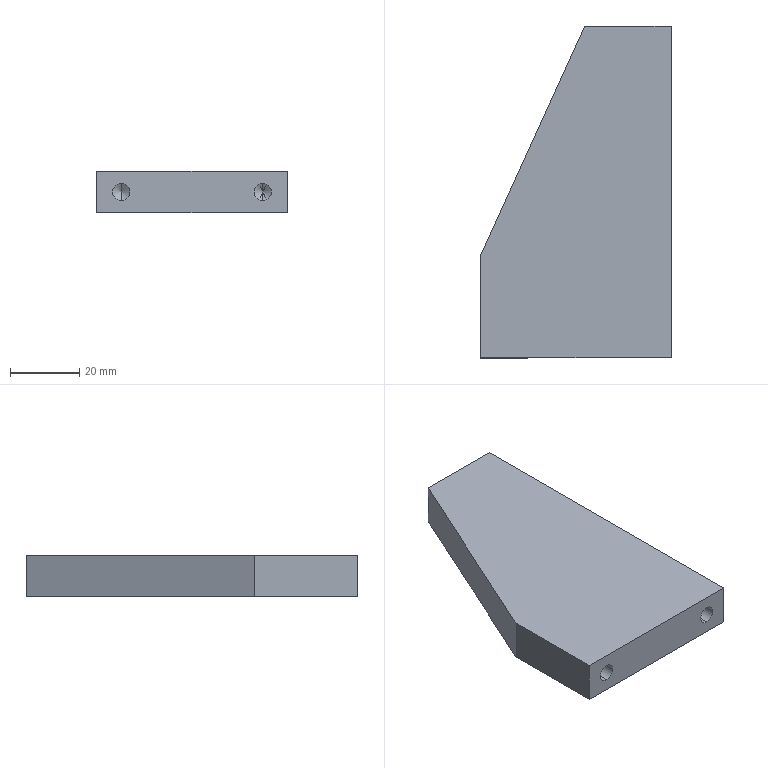Component | SolidWorks | ClampingAssembly-1_A83-1 | 1 solid | 23 faces | box 55 x 96 x 12 mm | volume 50263 mm3 | cylinder 8 | cone 8 | plane 7 | commonest cylinder face diameters 5 x8 | material A6061
build123d program:
from build123d import *

# Parameters (mm, degrees)
SKETCH1_W             = 96
SKETCH1_H             = 55
BOSS_EXTRUDE1_DEPTH   = 6
CUT_EXTRUDE1_DEPTH    = 57.606
M6_TAPPED_HOLE1_D     = 5
M6_TAPPED_HOLE1_DEPTH = 15
M6_TAPPED_HOLE1_TIP   = 1.502
M6_TAPPED_HOLE2_D     = 5
M6_TAPPED_HOLE2_DEPTH = 15
M6_TAPPED_HOLE2_TIP   = 1.502


with BuildPart() as part:
    # Sketch1 → Boss-Extrude1 (new, symmetric)
    with BuildSketch(Plane(origin=(0, 0, 0), x_dir=(0, 0, -1), z_dir=(1, 0, 0))):
        Rectangle(SKETCH1_W, SKETCH1_H)
    extrude(amount=BOSS_EXTRUDE1_DEPTH, both=True)

    # Sketch2 → Cut-Extrude1 (cut, through all)
    with BuildSketch(Plane(origin=(6, 0, 0), x_dir=(0, 0, -1), z_dir=(1, 0, 0))):
        Polygon((48, 27.5), (-18, 27.5), (48, -2.5), align=None)
    extrude(amount=-CUT_EXTRUDE1_DEPTH, mode=Mode.SUBTRACT)

    # M6 Tapped Hole1
    with Locations(Plane.XY.offset(48)):
        with Locations((0, -20.5), (0, 20.5)):
            Hole(M6_TAPPED_HOLE1_D / 2, depth=M6_TAPPED_HOLE1_DEPTH)
            with Locations((0, 0, -(M6_TAPPED_HOLE1_DEPTH + M6_TAPPED_HOLE1_TIP / 2))):  # 118° drill point
                Cone(0, M6_TAPPED_HOLE1_D / 2, M6_TAPPED_HOLE1_TIP, mode=Mode.SUBTRACT)

    # M6 Tapped Hole2
    with Locations(Plane(origin=(0, -27.5, 0), x_dir=(-1, 0, 0), z_dir=(0, -1, 0))):
        with Locations((0, -22), (0, 38)):
            Hole(M6_TAPPED_HOLE2_D / 2, depth=M6_TAPPED_HOLE2_DEPTH)
            with Locations((0, 0, -(M6_TAPPED_HOLE2_DEPTH + M6_TAPPED_HOLE2_TIP / 2))):  # 118° drill point
                Cone(0, M6_TAPPED_HOLE2_D / 2, M6_TAPPED_HOLE2_TIP, mode=Mode.SUBTRACT)


solid = part.part

# Placed as in the assembly
solid = solid.moved(Location((-57.051, 24.036, -0.5), (90, 0, 90)))
STEP:
#1=COLOUR_RGB('',0.7922,0.8196,0.9333);
#2=FILL_AREA_STYLE_COLOUR('',#1);
#3=FILL_AREA_STYLE('',(#2));
#4=SURFACE_STYLE_FILL_AREA(#3);
#5=SURFACE_SIDE_STYLE('',(#4));
#6=SURFACE_STYLE_USAGE(.BOTH.,#5);
#7=PRESENTATION_STYLE_ASSIGNMENT((#6));
#8=CARTESIAN_POINT('',(-1.754,-0.01828,-0.01969));
#9=VERTEX_POINT('',#8);
#10=CARTESIAN_POINT('',(-1.754,0.1786,-0.01969));
#11=VERTEX_POINT('',#10);
#12=CARTESIAN_POINT('',(-1.754,0.08015,-0.01969));
#13=DIRECTION('',(1.,0.,0.));
#14=DIRECTION('',(0.,1.,0.));
#15=AXIS2_PLACEMENT_3D('',#12,#13,#14);
#16=CIRCLE('',#15,0.09843);
#17=EDGE_CURVE('',#9,#11,#16,.T.);
#18=ORIENTED_EDGE('',*,*,#17,.F.);
#19=CARTESIAN_POINT('',(-1.163,-0.01828,-0.01969));
#20=VERTEX_POINT('',#19);
#21=CARTESIAN_POINT('',(-1.163,-0.01828,-0.01969));
#22=DIRECTION('',(1.,0.,0.));
#23=VECTOR('',#22,39.37);
#24=LINE('',#21,#23);
#25=EDGE_CURVE('',#9,#20,#24,.T.);
#26=ORIENTED_EDGE('',*,*,#25,.T.);
#27=CARTESIAN_POINT('',(-1.163,0.1786,-0.01969));
#28=VERTEX_POINT('',#27);
#29=CARTESIAN_POINT('',(-1.163,0.08015,-0.01969));
#30=DIRECTION('',(1.,0.,0.));
#31=DIRECTION('',(0.,1.,0.));
#32=AXIS2_PLACEMENT_3D('',#29,#30,#31);
#33=CIRCLE('',#32,0.09843);
#34=EDGE_CURVE('',#20,#28,#33,.T.);
#35=ORIENTED_EDGE('',*,*,#34,.T.);
#36=CARTESIAN_POINT('',(-1.163,0.1786,-0.01969));
#37=DIRECTION('',(1.,0.,0.));
#38=VECTOR('',#37,39.37);
#39=LINE('',#36,#38);
#40=EDGE_CURVE('',#11,#28,#39,.T.);
#41=ORIENTED_EDGE('',*,*,#40,.F.);
#42=EDGE_LOOP('',(#18,#26,#35,#41));
#43=FACE_OUTER_BOUND('',#42,.T.);
#44=CARTESIAN_POINT('',(-1.163,0.08015,-0.01969));
#45=DIRECTION('',(1.,0.,0.));
#46=DIRECTION('',(0.,1.,0.));
#47=AXIS2_PLACEMENT_3D('',#44,#45,#46);
#48=CYLINDRICAL_SURFACE('',#47,0.09843);
#49=ADVANCED_FACE('',(#43),#48,.F.);
#50=CARTESIAN_POINT('',(-1.813,0.08015,-0.01969));
#51=VERTEX_POINT('',#50);
#52=CARTESIAN_POINT('',(-1.754,0.1786,-0.01969));
#53=DIRECTION('',(0.515,0.8572,0.));
#54=VECTOR('',#53,39.37);
#55=LINE('',#52,#54);
#56=EDGE_CURVE('',#51,#11,#55,.T.);
#57=ORIENTED_EDGE('',*,*,#56,.F.);
#58=CARTESIAN_POINT('',(-1.754,-0.01828,-0.01969));
#59=DIRECTION('',(0.515,-0.8572,-0.));
#60=VECTOR('',#59,39.37);
#61=LINE('',#58,#60);
#62=EDGE_CURVE('',#51,#9,#61,.T.);
#63=ORIENTED_EDGE('',*,*,#62,.T.);
#64=ORIENTED_EDGE('',*,*,#17,.T.);
#65=EDGE_LOOP('',(#57,#63,#64));
#66=FACE_OUTER_BOUND('',#65,.T.);
#67=CARTESIAN_POINT('',(-1.754,0.08015,-0.01969));
#68=DIRECTION('',(1.,0.,0.));
#69=DIRECTION('',(0.,1.,0.));
#70=AXIS2_PLACEMENT_3D('',#67,#68,#69);
#71=CONICAL_SURFACE('',#70,0.09843,1.03);
#72=ADVANCED_FACE('',(#66),#71,.F.);
#73=CARTESIAN_POINT('',(-1.754,2.344,-0.01969));
#74=VERTEX_POINT('',#73);
#75=CARTESIAN_POINT('',(-1.754,2.541,-0.01969));
#76=VERTEX_POINT('',#75);
#77=CARTESIAN_POINT('',(-1.754,2.442,-0.01969));
#78=DIRECTION('',(1.,0.,0.));
#79=DIRECTION('',(0.,1.,0.));
#80=AXIS2_PLACEMENT_3D('',#77,#78,#79);
#81=CIRCLE('',#80,0.09843);
#82=EDGE_CURVE('',#74,#76,#81,.T.);
#83=ORIENTED_EDGE('',*,*,#82,.F.);
#84=CARTESIAN_POINT('',(-1.163,2.344,-0.01969));
#85=VERTEX_POINT('',#84);
#86=CARTESIAN_POINT('',(-1.163,2.344,-0.01969));
#87=DIRECTION('',(1.,0.,0.));
#88=VECTOR('',#87,39.37);
#89=LINE('',#86,#88);
#90=EDGE_CURVE('',#74,#85,#89,.T.);
#91=ORIENTED_EDGE('',*,*,#90,.T.);
#92=CARTESIAN_POINT('',(-1.163,2.541,-0.01969));
#93=VERTEX_POINT('',#92);
#94=CARTESIAN_POINT('',(-1.163,2.442,-0.01969));
#95=DIRECTION('',(1.,0.,0.));
#96=DIRECTION('',(0.,1.,0.));
#97=AXIS2_PLACEMENT_3D('',#94,#95,#96);
#98=CIRCLE('',#97,0.09843);
#99=EDGE_CURVE('',#85,#93,#98,.T.);
#100=ORIENTED_EDGE('',*,*,#99,.T.);
#101=CARTESIAN_POINT('',(-1.163,2.541,-0.01969));
#102=DIRECTION('',(1.,0.,0.));
#103=VECTOR('',#102,39.37);
#104=LINE('',#101,#103);
#105=EDGE_CURVE('',#76,#93,#104,.T.);
#106=ORIENTED_EDGE('',*,*,#105,.F.);
#107=EDGE_LOOP('',(#83,#91,#100,#106));
#108=FACE_OUTER_BOUND('',#107,.T.);
#109=CARTESIAN_POINT('',(-1.163,2.442,-0.01969));
#110=DIRECTION('',(1.,0.,0.));
#111=DIRECTION('',(0.,1.,0.));
#112=AXIS2_PLACEMENT_3D('',#109,#110,#111);
#113=CYLINDRICAL_SURFACE('',#112,0.09843);
#114=ADVANCED_FACE('',(#108),#113,.F.);
#115=CARTESIAN_POINT('',(-1.813,2.442,-0.01969));
#116=VERTEX_POINT('',#115);
#117=CARTESIAN_POINT('',(-1.754,2.541,-0.01969));
#118=DIRECTION('',(0.515,0.8572,0.));
#119=VECTOR('',#118,39.37);
#120=LINE('',#117,#119);
#121=EDGE_CURVE('',#116,#76,#120,.T.);
#122=ORIENTED_EDGE('',*,*,#121,.F.);
#123=CARTESIAN_POINT('',(-1.754,2.344,-0.01969));
#124=DIRECTION('',(0.515,-0.8572,-0.));
#125=VECTOR('',#124,39.37);
#126=LINE('',#123,#125);
#127=EDGE_CURVE('',#116,#74,#126,.T.);
#128=ORIENTED_EDGE('',*,*,#127,.T.);
#129=ORIENTED_EDGE('',*,*,#82,.T.);
#130=EDGE_LOOP('',(#122,#128,#129));
#131=FACE_OUTER_BOUND('',#130,.T.);
#132=CARTESIAN_POINT('',(-1.754,2.442,-0.01969));
#133=DIRECTION('',(1.,0.,0.));
#134=DIRECTION('',(0.,1.,0.));
#135=AXIS2_PLACEMENT_3D('',#132,#133,#134);
#136=CONICAL_SURFACE('',#135,0.09843,1.03);
#137=ADVANCED_FACE('',(#131),#136,.F.);
#138=CARTESIAN_POINT('',(-1.439,-0.3529,-0.1181));
#139=VERTEX_POINT('',#138);
#140=CARTESIAN_POINT('',(-1.439,-0.3529,0.07874));
#141=VERTEX_POINT('',#140);
#142=CARTESIAN_POINT('',(-1.439,-0.3529,-0.01969));
#143=DIRECTION('',(0.,-1.,-0.));
#144=DIRECTION('',(0.,-0.,1.));
#145=AXIS2_PLACEMENT_3D('',#142,#143,#144);
#146=CIRCLE('',#145,0.09843);
#147=EDGE_CURVE('',#139,#141,#146,.T.);
#148=ORIENTED_EDGE('',*,*,#147,.F.);
#149=CARTESIAN_POINT('',(-1.439,-0.9435,-0.1181));
#150=VERTEX_POINT('',#149);
#151=CARTESIAN_POINT('',(-1.439,-0.9435,-0.1181));
#152=DIRECTION('',(0.,-1.,-0.));
#153=VECTOR('',#152,39.37);
#154=LINE('',#151,#153);
#155=EDGE_CURVE('',#139,#150,#154,.T.);
#156=ORIENTED_EDGE('',*,*,#155,.T.);
#157=CARTESIAN_POINT('',(-1.439,-0.9435,0.07874));
#158=VERTEX_POINT('',#157);
#159=CARTESIAN_POINT('',(-1.439,-0.9435,-0.01969));
#160=DIRECTION('',(0.,-1.,-0.));
#161=DIRECTION('',(0.,-0.,1.));
#162=AXIS2_PLACEMENT_3D('',#159,#160,#161);
#163=CIRCLE('',#162,0.09843);
#164=EDGE_CURVE('',#150,#158,#163,.T.);
#165=ORIENTED_EDGE('',*,*,#164,.T.);
#166=CARTESIAN_POINT('',(-1.439,-0.9435,0.07874));
#167=DIRECTION('',(0.,-1.,-0.));
#168=VECTOR('',#167,39.37);
#169=LINE('',#166,#168);
#170=EDGE_CURVE('',#141,#158,#169,.T.);
#171=ORIENTED_EDGE('',*,*,#170,.F.);
#172=EDGE_LOOP('',(#148,#156,#165,#171));
#173=FACE_OUTER_BOUND('',#172,.T.);
#174=CARTESIAN_POINT('',(-1.439,-0.9435,-0.01969));
#175=DIRECTION('',(0.,-1.,-0.));
#176=DIRECTION('',(0.,-0.,1.));
#177=AXIS2_PLACEMENT_3D('',#174,#175,#176);
#178=CYLINDRICAL_SURFACE('',#177,0.09843);
#179=ADVANCED_FACE('',(#173),#178,.F.);
#180=CARTESIAN_POINT('',(-1.439,-0.2938,-0.01969));
#181=VERTEX_POINT('',#180);
#182=CARTESIAN_POINT('',(-1.439,-0.3529,0.07874));
#183=DIRECTION('',(-0.,-0.515,0.8572));
#184=VECTOR('',#183,39.37);
#185=LINE('',#182,#184);
#186=EDGE_CURVE('',#181,#141,#185,.T.);
#187=ORIENTED_EDGE('',*,*,#186,.F.);
#188=CARTESIAN_POINT('',(-1.439,-0.3529,-0.1181));
#189=DIRECTION('',(0.,-0.515,-0.8572));
#190=VECTOR('',#189,39.37);
#191=LINE('',#188,#190);
#192=EDGE_CURVE('',#181,#139,#191,.T.);
#193=ORIENTED_EDGE('',*,*,#192,.T.);
#194=ORIENTED_EDGE('',*,*,#147,.T.);
#195=EDGE_LOOP('',(#187,#193,#194));
#196=FACE_OUTER_BOUND('',#195,.T.);
#197=CARTESIAN_POINT('',(-1.439,-0.3529,-0.01969));
#198=DIRECTION('',(0.,-1.,-0.));
#199=DIRECTION('',(0.,-0.,1.));
#200=AXIS2_PLACEMENT_3D('',#197,#198,#199);
#201=CONICAL_SURFACE('',#200,0.09843,1.03);
#202=ADVANCED_FACE('',(#196),#201,.F.);
#203=CARTESIAN_POINT('',(-3.053,-0.3529,-0.1181));
#204=VERTEX_POINT('',#203);
#205=CARTESIAN_POINT('',(-3.053,-0.3529,0.07874));
#206=VERTEX_POINT('',#205);
#207=CARTESIAN_POINT('',(-3.053,-0.3529,-0.01969));
#208=DIRECTION('',(0.,-1.,-0.));
#209=DIRECTION('',(0.,-0.,1.));
#210=AXIS2_PLACEMENT_3D('',#207,#208,#209);
#211=CIRCLE('',#210,0.09843);
#212=EDGE_CURVE('',#204,#206,#211,.T.);
#213=ORIENTED_EDGE('',*,*,#212,.F.);
#214=CARTESIAN_POINT('',(-3.053,-0.9435,-0.1181));
#215=VERTEX_POINT('',#214);
#216=CARTESIAN_POINT('',(-3.053,-0.9435,-0.1181));
#217=DIRECTION('',(0.,-1.,-0.));
#218=VECTOR('',#217,39.37);
#219=LINE('',#216,#218);
#220=EDGE_CURVE('',#204,#215,#219,.T.);
#221=ORIENTED_EDGE('',*,*,#220,.T.);
#222=CARTESIAN_POINT('',(-3.053,-0.9435,0.07874));
#223=VERTEX_POINT('',#222);
#224=CARTESIAN_POINT('',(-3.053,-0.9435,-0.01969));
#225=DIRECTION('',(0.,-1.,-0.));
#226=DIRECTION('',(0.,-0.,1.));
#227=AXIS2_PLACEMENT_3D('',#224,#225,#226);
#228=CIRCLE('',#227,0.09843);
#229=EDGE_CURVE('',#215,#223,#228,.T.);
#230=ORIENTED_EDGE('',*,*,#229,.T.);
#231=CARTESIAN_POINT('',(-3.053,-0.9435,0.07874));
#232=DIRECTION('',(0.,-1.,-0.));
#233=VECTOR('',#232,39.37);
#234=LINE('',#231,#233);
#235=EDGE_CURVE('',#206,#223,#234,.T.);
#236=ORIENTED_EDGE('',*,*,#235,.F.);
#237=EDGE_LOOP('',(#213,#221,#230,#236));
#238=FACE_OUTER_BOUND('',#237,.T.);
#239=CARTESIAN_POINT('',(-3.053,-0.9435,-0.01969));
#240=DIRECTION('',(0.,-1.,-0.));
#241=DIRECTION('',(0.,-0.,1.));
#242=AXIS2_PLACEMENT_3D('',#239,#240,#241);
#243=CYLINDRICAL_SURFACE('',#242,0.09843);
#244=ADVANCED_FACE('',(#238),#243,.F.);
#245=CARTESIAN_POINT('',(-3.053,-0.2938,-0.01969));
#246=VERTEX_POINT('',#245);
#247=CARTESIAN_POINT('',(-3.053,-0.3529,0.07874));
#248=DIRECTION('',(-0.,-0.515,0.8572));
#249=VECTOR('',#248,39.37);
#250=LINE('',#247,#249);
#251=EDGE_CURVE('',#246,#206,#250,.T.);
#252=ORIENTED_EDGE('',*,*,#251,.F.);
#253=CARTESIAN_POINT('',(-3.053,-0.3529,-0.1181));
#254=DIRECTION('',(0.,-0.515,-0.8572));
#255=VECTOR('',#254,39.37);
#256=LINE('',#253,#255);
#257=EDGE_CURVE('',#246,#204,#256,.T.);
#258=ORIENTED_EDGE('',*,*,#257,.T.);
#259=ORIENTED_EDGE('',*,*,#212,.T.);
#260=EDGE_LOOP('',(#252,#258,#259));
#261=FACE_OUTER_BOUND('',#260,.T.);
#262=CARTESIAN_POINT('',(-3.053,-0.3529,-0.01969));
#263=DIRECTION('',(0.,-1.,-0.));
#264=DIRECTION('',(0.,-0.,1.));
#265=AXIS2_PLACEMENT_3D('',#262,#263,#264);
#266=CONICAL_SURFACE('',#265,0.09843,1.03);
#267=ADVANCED_FACE('',(#261),#266,.F.);
#268=CARTESIAN_POINT('',(-1.163,2.836,-0.2559));
#269=VERTEX_POINT('',#268);
#270=CARTESIAN_POINT('',(-2.148,2.836,-0.2559));
#271=VERTEX_POINT('',#270);
#272=CARTESIAN_POINT('',(-3.329,2.836,-0.2559));
#273=DIRECTION('',(-1.,-0.,-0.));
#274=VECTOR('',#273,39.37);
#275=LINE('',#272,#274);
#276=EDGE_CURVE('',#269,#271,#275,.T.);
#277=ORIENTED_EDGE('',*,*,#276,.T.);
#278=CARTESIAN_POINT('',(-2.148,2.836,0.2165));
#279=VERTEX_POINT('',#278);
#280=CARTESIAN_POINT('',(-2.148,2.836,-0.2559));
#281=DIRECTION('',(-0.,-0.,1.));
#282=VECTOR('',#281,39.37);
#283=LINE('',#280,#282);
#284=EDGE_CURVE('',#271,#279,#283,.T.);
#285=ORIENTED_EDGE('',*,*,#284,.T.);
#286=CARTESIAN_POINT('',(-1.163,2.836,0.2165));
#287=VERTEX_POINT('',#286);
#288=CARTESIAN_POINT('',(-3.329,2.836,0.2165));
#289=DIRECTION('',(-1.,-0.,-0.));
#290=VECTOR('',#289,39.37);
#291=LINE('',#288,#290);
#292=EDGE_CURVE('',#287,#279,#291,.T.);
#293=ORIENTED_EDGE('',*,*,#292,.F.);
#294=CARTESIAN_POINT('',(-1.163,2.836,0.2165));
#295=DIRECTION('',(0.,0.,-1.));
#296=VECTOR('',#295,39.37);
#297=LINE('',#294,#296);
#298=EDGE_CURVE('',#287,#269,#297,.T.);
#299=ORIENTED_EDGE('',*,*,#298,.T.);
#300=EDGE_LOOP('',(#277,#285,#293,#299));
#301=FACE_OUTER_BOUND('',#300,.T.);
#302=CARTESIAN_POINT('',(-3.329,2.836,0.2165));
#303=DIRECTION('',(0.,-1.,-0.));
#304=DIRECTION('',(-0.,-0.,1.));
#305=AXIS2_PLACEMENT_3D('',#302,#303,#304);
#306=PLANE('',#305);
#307=ADVANCED_FACE('',(#301),#306,.F.);
#308=CARTESIAN_POINT('',(-3.329,0.2376,0.2165));
#309=VERTEX_POINT('',#308);
#310=CARTESIAN_POINT('',(-3.329,-0.9435,0.2165));
#311=VERTEX_POINT('',#310);
#312=CARTESIAN_POINT('',(-3.329,-0.9435,0.2165));
#313=DIRECTION('',(0.,-1.,-0.));
#314=VECTOR('',#313,39.37);
#315=LINE('',#312,#314);
#316=EDGE_CURVE('',#309,#311,#315,.T.);
#317=ORIENTED_EDGE('',*,*,#316,.F.);
#318=CARTESIAN_POINT('',(-3.329,0.2376,-0.2559));
#319=VERTEX_POINT('',#318);
#320=CARTESIAN_POINT('',(-3.329,0.2376,-0.2559));
#321=DIRECTION('',(-0.,-0.,1.));
#322=VECTOR('',#321,39.37);
#323=LINE('',#320,#322);
#324=EDGE_CURVE('',#319,#309,#323,.T.);
#325=ORIENTED_EDGE('',*,*,#324,.F.);
#326=CARTESIAN_POINT('',(-3.329,-0.9435,-0.2559));
#327=VERTEX_POINT('',#326);
#328=CARTESIAN_POINT('',(-3.329,-0.9435,-0.2559));
#329=DIRECTION('',(0.,-1.,-0.));
#330=VECTOR('',#329,39.37);
#331=LINE('',#328,#330);
#332=EDGE_CURVE('',#319,#327,#331,.T.);
#333=ORIENTED_EDGE('',*,*,#332,.T.);
#334=CARTESIAN_POINT('',(-3.329,-0.9435,0.2165));
#335=DIRECTION('',(0.,0.,-1.));
#336=VECTOR('',#335,39.37);
#337=LINE('',#334,#336);
#338=EDGE_CURVE('',#311,#327,#337,.T.);
#339=ORIENTED_EDGE('',*,*,#338,.F.);
#340=EDGE_LOOP('',(#317,#325,#333,#339));
#341=FACE_OUTER_BOUND('',#340,.T.);
#342=CARTESIAN_POINT('',(-3.329,-0.9435,0.2165));
#343=DIRECTION('',(1.,0.,0.));
#344=DIRECTION('',(-0.,1.,0.));
#345=AXIS2_PLACEMENT_3D('',#342,#343,#344);
#346=PLANE('',#345);
#347=ADVANCED_FACE('',(#341),#346,.F.);
#348=CARTESIAN_POINT('',(-1.439,-0.9435,-0.01969));
#349=DIRECTION('',(0.,-1.,-0.));
#350=DIRECTION('',(0.,-0.,1.));
#351=AXIS2_PLACEMENT_3D('',#348,#349,#350);
#352=CIRCLE('',#351,0.09843);
#353=EDGE_CURVE('',#158,#150,#352,.T.);
#354=ORIENTED_EDGE('',*,*,#353,.F.);
#355=ORIENTED_EDGE('',*,*,#164,.F.);
#356=EDGE_LOOP('',(#354,#355));
#357=FACE_BOUND('',#356,.T.);
#358=CARTESIAN_POINT('',(-3.053,-0.9435,-0.01969));
#359=DIRECTION('',(0.,-1.,-0.));
#360=DIRECTION('',(0.,-0.,1.));
#361=AXIS2_PLACEMENT_3D('',#358,#359,#360);
#362=CIRCLE('',#361,0.09843);
#363=EDGE_CURVE('',#223,#215,#362,.T.);
#364=ORIENTED_EDGE('',*,*,#363,.F.);
#365=ORIENTED_EDGE('',*,*,#229,.F.);
#366=EDGE_LOOP('',(#364,#365));
#367=FACE_BOUND('',#366,.T.);
#368=CARTESIAN_POINT('',(-1.163,-0.9435,-0.2559));
#369=VERTEX_POINT('',#368);
#370=CARTESIAN_POINT('',(-3.329,-0.9435,-0.2559));
#371=DIRECTION('',(1.,0.,0.));
#372=VECTOR('',#371,39.37);
#373=LINE('',#370,#372);
#374=EDGE_CURVE('',#327,#369,#373,.T.);
#375=ORIENTED_EDGE('',*,*,#374,.T.);
#376=CARTESIAN_POINT('',(-1.163,-0.9435,0.2165));
#377=VERTEX_POINT('',#376);
#378=CARTESIAN_POINT('',(-1.163,-0.9435,0.2165));
#379=DIRECTION('',(0.,0.,-1.));
#380=VECTOR('',#379,39.37);
#381=LINE('',#378,#380);
#382=EDGE_CURVE('',#377,#369,#381,.T.);
#383=ORIENTED_EDGE('',*,*,#382,.F.);
#384=CARTESIAN_POINT('',(-3.329,-0.9435,0.2165));
#385=DIRECTION('',(1.,0.,0.));
#386=VECTOR('',#385,39.37);
#387=LINE('',#384,#386);
#388=EDGE_CURVE('',#311,#377,#387,.T.);
#389=ORIENTED_EDGE('',*,*,#388,.F.);
#390=ORIENTED_EDGE('',*,*,#338,.T.);
#391=EDGE_LOOP('',(#375,#383,#389,#390));
#392=FACE_OUTER_BOUND('',#391,.T.);
#393=CARTESIAN_POINT('',(-3.329,-0.9435,0.2165));
#394=DIRECTION('',(-0.,1.,0.));
#395=DIRECTION('',(-1.,-0.,-0.));
#396=AXIS2_PLACEMENT_3D('',#393,#394,#395);
#397=PLANE('',#396);
#398=ADVANCED_FACE('',(#357,#367,#392),#397,.F.);
#399=CARTESIAN_POINT('',(-1.163,0.08015,-0.01969));
#400=DIRECTION('',(1.,0.,0.));
#401=DIRECTION('',(0.,1.,0.));
#402=AXIS2_PLACEMENT_3D('',#399,#400,#401);
#403=CIRCLE('',#402,0.09843);
#404=EDGE_CURVE('',#28,#20,#403,.T.);
#405=ORIENTED_EDGE('',*,*,#404,.F.);
#406=ORIENTED_EDGE('',*,*,#34,.F.);
#407=EDGE_LOOP('',(#405,#406));
#408=FACE_BOUND('',#407,.T.);
#409=CARTESIAN_POINT('',(-1.163,2.442,-0.01969));
#410=DIRECTION('',(1.,0.,0.));
#411=DIRECTION('',(0.,1.,0.));
#412=AXIS2_PLACEMENT_3D('',#409,#410,#411);
#413=CIRCLE('',#412,0.09843);
#414=EDGE_CURVE('',#93,#85,#413,.T.);
#415=ORIENTED_EDGE('',*,*,#414,.F.);
#416=ORIENTED_EDGE('',*,*,#99,.F.);
#417=EDGE_LOOP('',(#415,#416));
#418=FACE_BOUND('',#417,.T.);
#419=CARTESIAN_POINT('',(-1.163,-0.9435,-0.2559));
#420=DIRECTION('',(-0.,1.,0.));
#421=VECTOR('',#420,39.37);
#422=LINE('',#419,#421);
#423=EDGE_CURVE('',#369,#269,#422,.T.);
#424=ORIENTED_EDGE('',*,*,#423,.T.);
#425=ORIENTED_EDGE('',*,*,#298,.F.);
#426=CARTESIAN_POINT('',(-1.163,-0.9435,0.2165));
#427=DIRECTION('',(-0.,1.,0.));
#428=VECTOR('',#427,39.37);
#429=LINE('',#426,#428);
#430=EDGE_CURVE('',#377,#287,#429,.T.);
#431=ORIENTED_EDGE('',*,*,#430,.F.);
#432=ORIENTED_EDGE('',*,*,#382,.T.);
#433=EDGE_LOOP('',(#424,#425,#431,#432));
#434=FACE_OUTER_BOUND('',#433,.T.);
#435=CARTESIAN_POINT('',(-1.163,-0.9435,0.2165));
#436=DIRECTION('',(-1.,-0.,-0.));
#437=DIRECTION('',(0.,-1.,-0.));
#438=AXIS2_PLACEMENT_3D('',#435,#436,#437);
#439=PLANE('',#438);
#440=ADVANCED_FACE('',(#408,#418,#434),#439,.F.);
#441=CARTESIAN_POINT('',(-3.329,0.2376,0.2165));
#442=DIRECTION('',(0.4138,0.9104,0.));
#443=VECTOR('',#442,39.37);
#444=LINE('',#441,#443);
#445=EDGE_CURVE('',#309,#279,#444,.T.);
#446=ORIENTED_EDGE('',*,*,#445,.F.);
#447=ORIENTED_EDGE('',*,*,#316,.T.);
#448=ORIENTED_EDGE('',*,*,#388,.T.);
#449=ORIENTED_EDGE('',*,*,#430,.T.);
#450=ORIENTED_EDGE('',*,*,#292,.T.);
#451=EDGE_LOOP('',(#446,#447,#448,#449,#450));
#452=FACE_OUTER_BOUND('',#451,.T.);
#453=CARTESIAN_POINT('',(-2.246,0.9463,0.2165));
#454=DIRECTION('',(-0.,-0.,1.));
#455=DIRECTION('',(-0.,1.,0.));
#456=AXIS2_PLACEMENT_3D('',#453,#454,#455);
#457=PLANE('',#456);
#458=ADVANCED_FACE('',(#452),#457,.T.);
#459=ORIENTED_EDGE('',*,*,#332,.F.);
#460=CARTESIAN_POINT('',(-3.329,0.2376,-0.2559));
#461=DIRECTION('',(0.4138,0.9104,0.));
#462=VECTOR('',#461,39.37);
#463=LINE('',#460,#462);
#464=EDGE_CURVE('',#319,#271,#463,.T.);
#465=ORIENTED_EDGE('',*,*,#464,.T.);
#466=ORIENTED_EDGE('',*,*,#276,.F.);
#467=ORIENTED_EDGE('',*,*,#423,.F.);
#468=ORIENTED_EDGE('',*,*,#374,.F.);
#469=EDGE_LOOP('',(#459,#465,#466,#467,#468));
#470=FACE_OUTER_BOUND('',#469,.T.);
#471=CARTESIAN_POINT('',(-2.246,0.9463,-0.2559));
#472=DIRECTION('',(-0.,-0.,1.));
#473=DIRECTION('',(-0.,1.,0.));
#474=AXIS2_PLACEMENT_3D('',#471,#472,#473);
#475=PLANE('',#474);
#476=ADVANCED_FACE('',(#470),#475,.F.);
#477=ORIENTED_EDGE('',*,*,#445,.T.);
#478=ORIENTED_EDGE('',*,*,#284,.F.);
#479=ORIENTED_EDGE('',*,*,#464,.F.);
#480=ORIENTED_EDGE('',*,*,#324,.T.);
#481=EDGE_LOOP('',(#477,#478,#479,#480));
#482=FACE_OUTER_BOUND('',#481,.T.);
#483=CARTESIAN_POINT('',(-3.329,0.2376,-0.2559));
#484=DIRECTION('',(0.9104,-0.4138,-0.));
#485=DIRECTION('',(0.4138,0.9104,0.));
#486=AXIS2_PLACEMENT_3D('',#483,#484,#485);
#487=PLANE('',#486);
#488=ADVANCED_FACE('',(#482),#487,.F.);
#489=ORIENTED_EDGE('',*,*,#257,.F.);
#490=ORIENTED_EDGE('',*,*,#251,.T.);
#491=CARTESIAN_POINT('',(-3.053,-0.3529,-0.01969));
#492=DIRECTION('',(0.,-1.,-0.));
#493=DIRECTION('',(0.,-0.,1.));
#494=AXIS2_PLACEMENT_3D('',#491,#492,#493);
#495=CIRCLE('',#494,0.09843);
#496=EDGE_CURVE('',#206,#204,#495,.T.);
#497=ORIENTED_EDGE('',*,*,#496,.T.);
#498=EDGE_LOOP('',(#489,#490,#497));
#499=FACE_OUTER_BOUND('',#498,.T.);
#500=CARTESIAN_POINT('',(-3.053,-0.3529,-0.01969));
#501=DIRECTION('',(0.,-1.,-0.));
#502=DIRECTION('',(0.,-0.,1.));
#503=AXIS2_PLACEMENT_3D('',#500,#501,#502);
#504=CONICAL_SURFACE('',#503,0.09843,1.03);
#505=ADVANCED_FACE('',(#499),#504,.F.);
#506=ORIENTED_EDGE('',*,*,#220,.F.);
#507=ORIENTED_EDGE('',*,*,#496,.F.);
#508=ORIENTED_EDGE('',*,*,#235,.T.);
#509=ORIENTED_EDGE('',*,*,#363,.T.);
#510=EDGE_LOOP('',(#506,#507,#508,#509));
#511=FACE_OUTER_BOUND('',#510,.T.);
#512=CARTESIAN_POINT('',(-3.053,-0.9435,-0.01969));
#513=DIRECTION('',(0.,-1.,-0.));
#514=DIRECTION('',(0.,-0.,1.));
#515=AXIS2_PLACEMENT_3D('',#512,#513,#514);
#516=CYLINDRICAL_SURFACE('',#515,0.09843);
#517=ADVANCED_FACE('',(#511),#516,.F.);
#518=ORIENTED_EDGE('',*,*,#192,.F.);
#519=ORIENTED_EDGE('',*,*,#186,.T.);
#520=CARTESIAN_POINT('',(-1.439,-0.3529,-0.01969));
#521=DIRECTION('',(0.,-1.,-0.));
#522=DIRECTION('',(0.,-0.,1.));
#523=AXIS2_PLACEMENT_3D('',#520,#521,#522);
#524=CIRCLE('',#523,0.09843);
#525=EDGE_CURVE('',#141,#139,#524,.T.);
#526=ORIENTED_EDGE('',*,*,#525,.T.);
#527=EDGE_LOOP('',(#518,#519,#526));
#528=FACE_OUTER_BOUND('',#527,.T.);
#529=CARTESIAN_POINT('',(-1.439,-0.3529,-0.01969));
#530=DIRECTION('',(0.,-1.,-0.));
#531=DIRECTION('',(0.,-0.,1.));
#532=AXIS2_PLACEMENT_3D('',#529,#530,#531);
#533=CONICAL_SURFACE('',#532,0.09843,1.03);
#534=ADVANCED_FACE('',(#528),#533,.F.);
#535=ORIENTED_EDGE('',*,*,#155,.F.);
#536=ORIENTED_EDGE('',*,*,#525,.F.);
#537=ORIENTED_EDGE('',*,*,#170,.T.);
#538=ORIENTED_EDGE('',*,*,#353,.T.);
#539=EDGE_LOOP('',(#535,#536,#537,#538));
#540=FACE_OUTER_BOUND('',#539,.T.);
#541=CARTESIAN_POINT('',(-1.439,-0.9435,-0.01969));
#542=DIRECTION('',(0.,-1.,-0.));
#543=DIRECTION('',(0.,-0.,1.));
#544=AXIS2_PLACEMENT_3D('',#541,#542,#543);
#545=CYLINDRICAL_SURFACE('',#544,0.09843);
#546=ADVANCED_FACE('',(#540),#545,.F.);
#547=ORIENTED_EDGE('',*,*,#127,.F.);
#548=ORIENTED_EDGE('',*,*,#121,.T.);
#549=CARTESIAN_POINT('',(-1.754,2.442,-0.01969));
#550=DIRECTION('',(1.,0.,0.));
#551=DIRECTION('',(0.,1.,0.));
#552=AXIS2_PLACEMENT_3D('',#549,#550,#551);
#553=CIRCLE('',#552,0.09843);
#554=EDGE_CURVE('',#76,#74,#553,.T.);
#555=ORIENTED_EDGE('',*,*,#554,.T.);
#556=EDGE_LOOP('',(#547,#548,#555));
#557=FACE_OUTER_BOUND('',#556,.T.);
#558=CARTESIAN_POINT('',(-1.754,2.442,-0.01969));
#559=DIRECTION('',(1.,0.,0.));
#560=DIRECTION('',(0.,1.,0.));
#561=AXIS2_PLACEMENT_3D('',#558,#559,#560);
#562=CONICAL_SURFACE('',#561,0.09843,1.03);
#563=ADVANCED_FACE('',(#557),#562,.F.);
#564=ORIENTED_EDGE('',*,*,#90,.F.);
#565=ORIENTED_EDGE('',*,*,#554,.F.);
#566=ORIENTED_EDGE('',*,*,#105,.T.);
#567=ORIENTED_EDGE('',*,*,#414,.T.);
#568=EDGE_LOOP('',(#564,#565,#566,#567));
#569=FACE_OUTER_BOUND('',#568,.T.);
#570=CARTESIAN_POINT('',(-1.163,2.442,-0.01969));
#571=DIRECTION('',(1.,0.,0.));
#572=DIRECTION('',(0.,1.,0.));
#573=AXIS2_PLACEMENT_3D('',#570,#571,#572);
#574=CYLINDRICAL_SURFACE('',#573,0.09843);
#575=ADVANCED_FACE('',(#569),#574,.F.);
#576=ORIENTED_EDGE('',*,*,#62,.F.);
#577=ORIENTED_EDGE('',*,*,#56,.T.);
#578=CARTESIAN_POINT('',(-1.754,0.08015,-0.01969));
#579=DIRECTION('',(1.,0.,0.));
#580=DIRECTION('',(0.,1.,0.));
#581=AXIS2_PLACEMENT_3D('',#578,#579,#580);
#582=CIRCLE('',#581,0.09843);
#583=EDGE_CURVE('',#11,#9,#582,.T.);
#584=ORIENTED_EDGE('',*,*,#583,.T.);
#585=EDGE_LOOP('',(#576,#577,#584));
#586=FACE_OUTER_BOUND('',#585,.T.);
#587=CARTESIAN_POINT('',(-1.754,0.08015,-0.01969));
#588=DIRECTION('',(1.,0.,0.));
#589=DIRECTION('',(0.,1.,0.));
#590=AXIS2_PLACEMENT_3D('',#587,#588,#589);
#591=CONICAL_SURFACE('',#590,0.09843,1.03);
#592=ADVANCED_FACE('',(#586),#591,.F.);
#593=ORIENTED_EDGE('',*,*,#25,.F.);
#594=ORIENTED_EDGE('',*,*,#583,.F.);
#595=ORIENTED_EDGE('',*,*,#40,.T.);
#596=ORIENTED_EDGE('',*,*,#404,.T.);
#597=EDGE_LOOP('',(#593,#594,#595,#596));
#598=FACE_OUTER_BOUND('',#597,.T.);
#599=CARTESIAN_POINT('',(-1.163,0.08015,-0.01969));
#600=DIRECTION('',(1.,0.,0.));
#601=DIRECTION('',(0.,1.,0.));
#602=AXIS2_PLACEMENT_3D('',#599,#600,#601);
#603=CYLINDRICAL_SURFACE('',#602,0.09843);
#604=ADVANCED_FACE('',(#598),#603,.F.);
#605=CLOSED_SHELL('',(#49,#72,#114,#137,#179,#202,#244,#267,#307,#347,#398,#440,#458,#476,#488,#505,#517,#534,#546,#563,#575,#592,#604));
#606=MANIFOLD_SOLID_BREP('',#605);
#607=STYLED_ITEM('',(#7),#606);
#608=(LENGTH_UNIT()NAMED_UNIT(*)SI_UNIT($,.METRE.));
#609=LENGTH_MEASURE_WITH_UNIT(LENGTH_MEASURE(0.0254),#608);
#610=DIMENSIONAL_EXPONENTS(1.,0.,0.,0.,0.,0.,0.);
#611=(CONVERSION_BASED_UNIT('',#609)LENGTH_UNIT()NAMED_UNIT(#610));
#612=UNCERTAINTY_MEASURE_WITH_UNIT(LENGTH_MEASURE(0.00001),#611,'','');
#613=(NAMED_UNIT(*)PLANE_ANGLE_UNIT()SI_UNIT($,.RADIAN.));
#614=(NAMED_UNIT(*)SI_UNIT($,.STERADIAN.)SOLID_ANGLE_UNIT());
#615=(GEOMETRIC_REPRESENTATION_CONTEXT(3)GLOBAL_UNCERTAINTY_ASSIGNED_CONTEXT((#612))GLOBAL_UNIT_ASSIGNED_CONTEXT((#611,#613,#614))REPRESENTATION_CONTEXT('',''));
#616=MECHANICAL_DESIGN_GEOMETRIC_PRESENTATION_REPRESENTATION('',(#607),#615);
#617=CARTESIAN_POINT('',(0.,0.,0.));
#618=DIRECTION('',(0.,0.,1.));
#619=DIRECTION('',(1.,0.,0.));
#620=AXIS2_PLACEMENT_3D('',#617,#618,#619);
#621=(LENGTH_UNIT()NAMED_UNIT(*)SI_UNIT($,.METRE.));
#622=LENGTH_MEASURE_WITH_UNIT(LENGTH_MEASURE(0.0254),#621);
#623=DIMENSIONAL_EXPONENTS(1.,0.,0.,0.,0.,0.,0.);
#624=(CONVERSION_BASED_UNIT('',#622)LENGTH_UNIT()NAMED_UNIT(#623));
#625=UNCERTAINTY_MEASURE_WITH_UNIT(LENGTH_MEASURE(0.00001),#624,'','');
#626=(NAMED_UNIT(*)PLANE_ANGLE_UNIT()SI_UNIT($,.RADIAN.));
#627=(NAMED_UNIT(*)SI_UNIT($,.STERADIAN.)SOLID_ANGLE_UNIT());
#628=(GEOMETRIC_REPRESENTATION_CONTEXT(3)GLOBAL_UNCERTAINTY_ASSIGNED_CONTEXT((#625))GLOBAL_UNIT_ASSIGNED_CONTEXT((#624,#626,#627))REPRESENTATION_CONTEXT('',''));
#629=ADVANCED_BREP_SHAPE_REPRESENTATION('',(#606,#620),#628);
#630=PRESENTATION_LAYER_ASSIGNMENT('','',(#607));